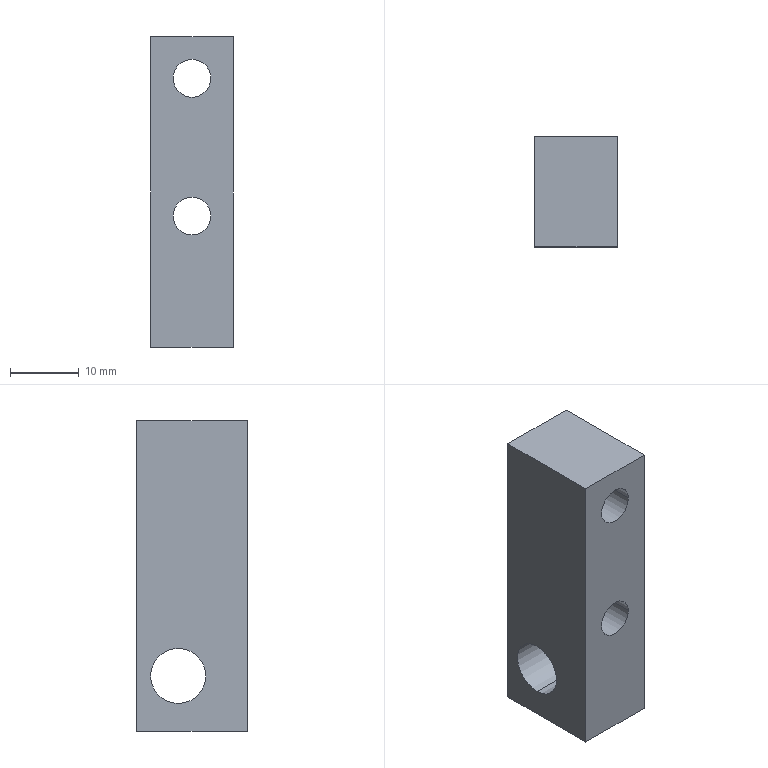Component | SolidWorks | STB-08-008-3 | 1 solid | 12 faces | box 12 x 16 x 45 mm | volume 7277 mm3 | cylinder 6 | plane 6 | commonest cylinder face diameters 5.5 x4 8 x2
build123d program:
from build123d import *

# Parameters (mm, degrees)
SKETCH1_W                  = 45
SKETCH1_H                  = 16
BOSS_EXTRUDE1_DEPTH        = 6
CUT_EXTRUDE1_REACH         = 28.725
SKETCH2_R                  = 4
F_5_5_5_5_DIAMETER_HOLE1_D = 5.5


with BuildPart() as part:
    # Sketch1 → Boss-Extrude1 (new, symmetric)
    with BuildSketch(Plane.XY):
        Rectangle(SKETCH1_W, SKETCH1_H)
    extrude(amount=BOSS_EXTRUDE1_DEPTH, both=True)

    # Sketch2 → Cut-Extrude1 (cut, up to next)
    with BuildSketch(Plane(origin=(0, 0, -6), x_dir=(-1, 0, 0), z_dir=(0, 0, -1)), mode=Mode.PRIVATE) as cut_extrude1_sk1:
        with Locations((14.5, 2)):
            Circle(SKETCH2_R)
    cut_extrude1_tool1 = extrude(cut_extrude1_sk1.sketch, amount=-CUT_EXTRUDE1_REACH, mode=Mode.PRIVATE) & part.part
    add(cut_extrude1_tool1.solids().sort_by_distance((-14.5, 2, -6))[0], mode=Mode.SUBTRACT)

    # 5.5 _5.5_ Diameter Hole1 (through all)
    with Locations(Plane(origin=(0, 8, 0), x_dir=(-1, 0, 0), z_dir=(0, 1, 0))):
        with Locations((-16.5, 0), (3.5, 0)):
            Hole(F_5_5_5_5_DIAMETER_HOLE1_D / 2)


solid = part.part

# Placed as in the assembly
solid = solid.moved(Location((-232.904, 163.999, -4.5), (0, -90, 0)))
STEP:
#1=CARTESIAN_POINT('',(-9.061,6.142,0.4724));
#2=VERTEX_POINT('',#1);
#3=CARTESIAN_POINT('',(-9.278,6.142,0.4724));
#4=VERTEX_POINT('',#3);
#5=CARTESIAN_POINT('',(-9.169,6.142,0.4724));
#6=DIRECTION('',(0.,1.,-0.));
#7=DIRECTION('',(0.,0.,-1.));
#8=AXIS2_PLACEMENT_3D('',#5,#6,#7);
#9=CIRCLE('',#8,0.1083);
#10=EDGE_CURVE('',#2,#4,#9,.T.);
#11=ORIENTED_EDGE('',*,*,#10,.F.);
#12=CARTESIAN_POINT('',(-9.061,6.772,0.4724));
#13=VERTEX_POINT('',#12);
#14=CARTESIAN_POINT('',(-9.061,6.772,0.4724));
#15=DIRECTION('',(0.,1.,0.));
#16=VECTOR('',#15,39.37);
#17=LINE('',#14,#16);
#18=EDGE_CURVE('',#2,#13,#17,.T.);
#19=ORIENTED_EDGE('',*,*,#18,.T.);
#20=CARTESIAN_POINT('',(-9.278,6.772,0.4724));
#21=VERTEX_POINT('',#20);
#22=CARTESIAN_POINT('',(-9.169,6.772,0.4724));
#23=DIRECTION('',(0.,1.,0.));
#24=DIRECTION('',(-1.,0.,-0.));
#25=AXIS2_PLACEMENT_3D('',#22,#23,#24);
#26=CIRCLE('',#25,0.1083);
#27=EDGE_CURVE('',#13,#21,#26,.T.);
#28=ORIENTED_EDGE('',*,*,#27,.T.);
#29=CARTESIAN_POINT('',(-9.278,6.772,0.4724));
#30=DIRECTION('',(0.,1.,0.));
#31=VECTOR('',#30,39.37);
#32=LINE('',#29,#31);
#33=EDGE_CURVE('',#4,#21,#32,.T.);
#34=ORIENTED_EDGE('',*,*,#33,.F.);
#35=EDGE_LOOP('',(#11,#19,#28,#34));
#36=FACE_OUTER_BOUND('',#35,.T.);
#37=CARTESIAN_POINT('',(-9.169,6.772,0.4724));
#38=DIRECTION('',(0.,1.,0.));
#39=DIRECTION('',(-1.,0.,-0.));
#40=AXIS2_PLACEMENT_3D('',#37,#38,#39);
#41=CYLINDRICAL_SURFACE('',#40,0.1083);
#42=ADVANCED_FACE('',(#36),#41,.F.);
#43=CARTESIAN_POINT('',(-9.061,6.142,-0.315));
#44=VERTEX_POINT('',#43);
#45=CARTESIAN_POINT('',(-9.278,6.142,-0.315));
#46=VERTEX_POINT('',#45);
#47=CARTESIAN_POINT('',(-9.169,6.142,-0.315));
#48=DIRECTION('',(0.,1.,-0.));
#49=DIRECTION('',(0.,0.,-1.));
#50=AXIS2_PLACEMENT_3D('',#47,#48,#49);
#51=CIRCLE('',#50,0.1083);
#52=EDGE_CURVE('',#44,#46,#51,.T.);
#53=ORIENTED_EDGE('',*,*,#52,.F.);
#54=CARTESIAN_POINT('',(-9.061,6.772,-0.315));
#55=VERTEX_POINT('',#54);
#56=CARTESIAN_POINT('',(-9.061,6.772,-0.315));
#57=DIRECTION('',(0.,1.,0.));
#58=VECTOR('',#57,39.37);
#59=LINE('',#56,#58);
#60=EDGE_CURVE('',#44,#55,#59,.T.);
#61=ORIENTED_EDGE('',*,*,#60,.T.);
#62=CARTESIAN_POINT('',(-9.278,6.772,-0.315));
#63=VERTEX_POINT('',#62);
#64=CARTESIAN_POINT('',(-9.169,6.772,-0.315));
#65=DIRECTION('',(0.,1.,0.));
#66=DIRECTION('',(-1.,0.,-0.));
#67=AXIS2_PLACEMENT_3D('',#64,#65,#66);
#68=CIRCLE('',#67,0.1083);
#69=EDGE_CURVE('',#55,#63,#68,.T.);
#70=ORIENTED_EDGE('',*,*,#69,.T.);
#71=CARTESIAN_POINT('',(-9.278,6.772,-0.315));
#72=DIRECTION('',(0.,1.,0.));
#73=VECTOR('',#72,39.37);
#74=LINE('',#71,#73);
#75=EDGE_CURVE('',#46,#63,#74,.T.);
#76=ORIENTED_EDGE('',*,*,#75,.F.);
#77=EDGE_LOOP('',(#53,#61,#70,#76));
#78=FACE_OUTER_BOUND('',#77,.T.);
#79=CARTESIAN_POINT('',(-9.169,6.772,-0.315));
#80=DIRECTION('',(0.,1.,0.));
#81=DIRECTION('',(-1.,0.,-0.));
#82=AXIS2_PLACEMENT_3D('',#79,#80,#81);
#83=CYLINDRICAL_SURFACE('',#82,0.1083);
#84=ADVANCED_FACE('',(#78),#83,.F.);
#85=CARTESIAN_POINT('',(-9.406,6.535,-0.5906));
#86=VERTEX_POINT('',#85);
#87=CARTESIAN_POINT('',(-9.406,6.535,-0.9055));
#88=VERTEX_POINT('',#87);
#89=CARTESIAN_POINT('',(-9.406,6.535,-0.748));
#90=DIRECTION('',(1.,0.,0.));
#91=DIRECTION('',(0.,0.,1.));
#92=AXIS2_PLACEMENT_3D('',#89,#90,#91);
#93=CIRCLE('',#92,0.1575);
#94=EDGE_CURVE('',#86,#88,#93,.T.);
#95=ORIENTED_EDGE('',*,*,#94,.F.);
#96=CARTESIAN_POINT('',(-8.933,6.535,-0.5906));
#97=VERTEX_POINT('',#96);
#98=CARTESIAN_POINT('',(-9.406,6.535,-0.5906));
#99=DIRECTION('',(1.,0.,0.));
#100=VECTOR('',#99,39.37);
#101=LINE('',#98,#100);
#102=EDGE_CURVE('',#86,#97,#101,.T.);
#103=ORIENTED_EDGE('',*,*,#102,.T.);
#104=CARTESIAN_POINT('',(-8.933,6.535,-0.9055));
#105=VERTEX_POINT('',#104);
#106=CARTESIAN_POINT('',(-8.933,6.535,-0.748));
#107=DIRECTION('',(1.,0.,0.));
#108=DIRECTION('',(0.,0.,-1.));
#109=AXIS2_PLACEMENT_3D('',#106,#107,#108);
#110=CIRCLE('',#109,0.1575);
#111=EDGE_CURVE('',#97,#105,#110,.T.);
#112=ORIENTED_EDGE('',*,*,#111,.T.);
#113=CARTESIAN_POINT('',(-9.406,6.535,-0.9055));
#114=DIRECTION('',(1.,0.,0.));
#115=VECTOR('',#114,39.37);
#116=LINE('',#113,#115);
#117=EDGE_CURVE('',#88,#105,#116,.T.);
#118=ORIENTED_EDGE('',*,*,#117,.F.);
#119=EDGE_LOOP('',(#95,#103,#112,#118));
#120=FACE_OUTER_BOUND('',#119,.T.);
#121=CARTESIAN_POINT('',(-9.406,6.535,-0.748));
#122=DIRECTION('',(1.,0.,0.));
#123=DIRECTION('',(0.,0.,-1.));
#124=AXIS2_PLACEMENT_3D('',#121,#122,#123);
#125=CYLINDRICAL_SURFACE('',#124,0.1575);
#126=ADVANCED_FACE('',(#120),#125,.F.);
#127=CARTESIAN_POINT('',(-8.933,6.772,-1.063));
#128=VERTEX_POINT('',#127);
#129=CARTESIAN_POINT('',(-8.933,6.142,-1.063));
#130=VERTEX_POINT('',#129);
#131=CARTESIAN_POINT('',(-8.933,6.772,-1.063));
#132=DIRECTION('',(-0.,-1.,-0.));
#133=VECTOR('',#132,39.37);
#134=LINE('',#131,#133);
#135=EDGE_CURVE('',#128,#130,#134,.T.);
#136=ORIENTED_EDGE('',*,*,#135,.T.);
#137=CARTESIAN_POINT('',(-9.406,6.142,-1.063));
#138=VERTEX_POINT('',#137);
#139=CARTESIAN_POINT('',(-9.406,6.142,-1.063));
#140=DIRECTION('',(1.,0.,0.));
#141=VECTOR('',#140,39.37);
#142=LINE('',#139,#141);
#143=EDGE_CURVE('',#138,#130,#142,.T.);
#144=ORIENTED_EDGE('',*,*,#143,.F.);
#145=CARTESIAN_POINT('',(-9.406,6.772,-1.063));
#146=VERTEX_POINT('',#145);
#147=CARTESIAN_POINT('',(-9.406,6.772,-1.063));
#148=DIRECTION('',(-0.,-1.,-0.));
#149=VECTOR('',#148,39.37);
#150=LINE('',#147,#149);
#151=EDGE_CURVE('',#146,#138,#150,.T.);
#152=ORIENTED_EDGE('',*,*,#151,.F.);
#153=CARTESIAN_POINT('',(-9.406,6.772,-1.063));
#154=DIRECTION('',(1.,0.,0.));
#155=VECTOR('',#154,39.37);
#156=LINE('',#153,#155);
#157=EDGE_CURVE('',#146,#128,#156,.T.);
#158=ORIENTED_EDGE('',*,*,#157,.T.);
#159=EDGE_LOOP('',(#136,#144,#152,#158));
#160=FACE_OUTER_BOUND('',#159,.T.);
#161=CARTESIAN_POINT('',(-9.406,6.772,-1.063));
#162=DIRECTION('',(-0.,-0.,1.));
#163=DIRECTION('',(1.,0.,0.));
#164=AXIS2_PLACEMENT_3D('',#161,#162,#163);
#165=PLANE('',#164);
#166=ADVANCED_FACE('',(#160),#165,.F.);
#167=CARTESIAN_POINT('',(-9.169,6.142,0.4724));
#168=DIRECTION('',(0.,1.,-0.));
#169=DIRECTION('',(0.,0.,-1.));
#170=AXIS2_PLACEMENT_3D('',#167,#168,#169);
#171=CIRCLE('',#170,0.1083);
#172=EDGE_CURVE('',#4,#2,#171,.T.);
#173=ORIENTED_EDGE('',*,*,#172,.T.);
#174=ORIENTED_EDGE('',*,*,#10,.T.);
#175=EDGE_LOOP('',(#173,#174));
#176=FACE_BOUND('',#175,.T.);
#177=CARTESIAN_POINT('',(-9.169,6.142,-0.315));
#178=DIRECTION('',(0.,1.,-0.));
#179=DIRECTION('',(0.,0.,-1.));
#180=AXIS2_PLACEMENT_3D('',#177,#178,#179);
#181=CIRCLE('',#180,0.1083);
#182=EDGE_CURVE('',#46,#44,#181,.T.);
#183=ORIENTED_EDGE('',*,*,#182,.T.);
#184=ORIENTED_EDGE('',*,*,#52,.T.);
#185=EDGE_LOOP('',(#183,#184));
#186=FACE_BOUND('',#185,.T.);
#187=CARTESIAN_POINT('',(-8.933,6.142,0.7087));
#188=VERTEX_POINT('',#187);
#189=CARTESIAN_POINT('',(-8.933,6.142,-1.063));
#190=DIRECTION('',(-0.,-0.,1.));
#191=VECTOR('',#190,39.37);
#192=LINE('',#189,#191);
#193=EDGE_CURVE('',#130,#188,#192,.T.);
#194=ORIENTED_EDGE('',*,*,#193,.T.);
#195=CARTESIAN_POINT('',(-9.406,6.142,0.7087));
#196=VERTEX_POINT('',#195);
#197=CARTESIAN_POINT('',(-9.406,6.142,0.7087));
#198=DIRECTION('',(1.,0.,0.));
#199=VECTOR('',#198,39.37);
#200=LINE('',#197,#199);
#201=EDGE_CURVE('',#196,#188,#200,.T.);
#202=ORIENTED_EDGE('',*,*,#201,.F.);
#203=CARTESIAN_POINT('',(-9.406,6.142,-1.063));
#204=DIRECTION('',(-0.,-0.,1.));
#205=VECTOR('',#204,39.37);
#206=LINE('',#203,#205);
#207=EDGE_CURVE('',#138,#196,#206,.T.);
#208=ORIENTED_EDGE('',*,*,#207,.F.);
#209=ORIENTED_EDGE('',*,*,#143,.T.);
#210=EDGE_LOOP('',(#194,#202,#208,#209));
#211=FACE_OUTER_BOUND('',#210,.T.);
#212=CARTESIAN_POINT('',(-9.406,6.142,-1.063));
#213=DIRECTION('',(0.,1.,0.));
#214=DIRECTION('',(0.,0.,-1.));
#215=AXIS2_PLACEMENT_3D('',#212,#213,#214);
#216=PLANE('',#215);
#217=ADVANCED_FACE('',(#176,#186,#211),#216,.F.);
#218=CARTESIAN_POINT('',(-8.933,6.772,0.7087));
#219=VERTEX_POINT('',#218);
#220=CARTESIAN_POINT('',(-8.933,6.772,0.7087));
#221=DIRECTION('',(0.,1.,0.));
#222=VECTOR('',#221,39.37);
#223=LINE('',#220,#222);
#224=EDGE_CURVE('',#188,#219,#223,.T.);
#225=ORIENTED_EDGE('',*,*,#224,.T.);
#226=CARTESIAN_POINT('',(-9.406,6.772,0.7087));
#227=VERTEX_POINT('',#226);
#228=CARTESIAN_POINT('',(-9.406,6.772,0.7087));
#229=DIRECTION('',(1.,0.,0.));
#230=VECTOR('',#229,39.37);
#231=LINE('',#228,#230);
#232=EDGE_CURVE('',#227,#219,#231,.T.);
#233=ORIENTED_EDGE('',*,*,#232,.F.);
#234=CARTESIAN_POINT('',(-9.406,6.772,0.7087));
#235=DIRECTION('',(0.,1.,0.));
#236=VECTOR('',#235,39.37);
#237=LINE('',#234,#236);
#238=EDGE_CURVE('',#196,#227,#237,.T.);
#239=ORIENTED_EDGE('',*,*,#238,.F.);
#240=ORIENTED_EDGE('',*,*,#201,.T.);
#241=EDGE_LOOP('',(#225,#233,#239,#240));
#242=FACE_OUTER_BOUND('',#241,.T.);
#243=CARTESIAN_POINT('',(-9.406,6.772,0.7087));
#244=DIRECTION('',(0.,0.,-1.));
#245=DIRECTION('',(-1.,-0.,-0.));
#246=AXIS2_PLACEMENT_3D('',#243,#244,#245);
#247=PLANE('',#246);
#248=ADVANCED_FACE('',(#242),#247,.F.);
#249=CARTESIAN_POINT('',(-9.169,6.772,0.4724));
#250=DIRECTION('',(0.,1.,0.));
#251=DIRECTION('',(-1.,0.,-0.));
#252=AXIS2_PLACEMENT_3D('',#249,#250,#251);
#253=CIRCLE('',#252,0.1083);
#254=EDGE_CURVE('',#21,#13,#253,.T.);
#255=ORIENTED_EDGE('',*,*,#254,.F.);
#256=ORIENTED_EDGE('',*,*,#27,.F.);
#257=EDGE_LOOP('',(#255,#256));
#258=FACE_BOUND('',#257,.T.);
#259=CARTESIAN_POINT('',(-9.169,6.772,-0.315));
#260=DIRECTION('',(0.,1.,0.));
#261=DIRECTION('',(-1.,0.,-0.));
#262=AXIS2_PLACEMENT_3D('',#259,#260,#261);
#263=CIRCLE('',#262,0.1083);
#264=EDGE_CURVE('',#63,#55,#263,.T.);
#265=ORIENTED_EDGE('',*,*,#264,.F.);
#266=ORIENTED_EDGE('',*,*,#69,.F.);
#267=EDGE_LOOP('',(#265,#266));
#268=FACE_BOUND('',#267,.T.);
#269=CARTESIAN_POINT('',(-8.933,6.772,-1.063));
#270=DIRECTION('',(0.,0.,-1.));
#271=VECTOR('',#270,39.37);
#272=LINE('',#269,#271);
#273=EDGE_CURVE('',#219,#128,#272,.T.);
#274=ORIENTED_EDGE('',*,*,#273,.T.);
#275=ORIENTED_EDGE('',*,*,#157,.F.);
#276=CARTESIAN_POINT('',(-9.406,6.772,-1.063));
#277=DIRECTION('',(0.,0.,-1.));
#278=VECTOR('',#277,39.37);
#279=LINE('',#276,#278);
#280=EDGE_CURVE('',#227,#146,#279,.T.);
#281=ORIENTED_EDGE('',*,*,#280,.F.);
#282=ORIENTED_EDGE('',*,*,#232,.T.);
#283=EDGE_LOOP('',(#274,#275,#281,#282));
#284=FACE_OUTER_BOUND('',#283,.T.);
#285=CARTESIAN_POINT('',(-9.406,6.772,-1.063));
#286=DIRECTION('',(0.,-1.,-0.));
#287=DIRECTION('',(1.,0.,0.));
#288=AXIS2_PLACEMENT_3D('',#285,#286,#287);
#289=PLANE('',#288);
#290=ADVANCED_FACE('',(#258,#268,#284),#289,.F.);
#291=CARTESIAN_POINT('',(-9.406,6.535,-0.748));
#292=DIRECTION('',(1.,0.,0.));
#293=DIRECTION('',(0.,0.,1.));
#294=AXIS2_PLACEMENT_3D('',#291,#292,#293);
#295=CIRCLE('',#294,0.1575);
#296=EDGE_CURVE('',#88,#86,#295,.T.);
#297=ORIENTED_EDGE('',*,*,#296,.T.);
#298=ORIENTED_EDGE('',*,*,#94,.T.);
#299=EDGE_LOOP('',(#297,#298));
#300=FACE_BOUND('',#299,.T.);
#301=ORIENTED_EDGE('',*,*,#151,.T.);
#302=ORIENTED_EDGE('',*,*,#207,.T.);
#303=ORIENTED_EDGE('',*,*,#238,.T.);
#304=ORIENTED_EDGE('',*,*,#280,.T.);
#305=EDGE_LOOP('',(#301,#302,#303,#304));
#306=FACE_OUTER_BOUND('',#305,.T.);
#307=CARTESIAN_POINT('',(-9.406,6.142,-1.063));
#308=DIRECTION('',(-1.,-0.,-0.));
#309=DIRECTION('',(-0.,-0.,1.));
#310=AXIS2_PLACEMENT_3D('',#307,#308,#309);
#311=PLANE('',#310);
#312=ADVANCED_FACE('',(#300,#306),#311,.T.);
#313=CARTESIAN_POINT('',(-8.933,6.535,-0.748));
#314=DIRECTION('',(1.,0.,0.));
#315=DIRECTION('',(0.,0.,-1.));
#316=AXIS2_PLACEMENT_3D('',#313,#314,#315);
#317=CIRCLE('',#316,0.1575);
#318=EDGE_CURVE('',#105,#97,#317,.T.);
#319=ORIENTED_EDGE('',*,*,#318,.F.);
#320=ORIENTED_EDGE('',*,*,#111,.F.);
#321=EDGE_LOOP('',(#319,#320));
#322=FACE_BOUND('',#321,.T.);
#323=ORIENTED_EDGE('',*,*,#135,.F.);
#324=ORIENTED_EDGE('',*,*,#273,.F.);
#325=ORIENTED_EDGE('',*,*,#224,.F.);
#326=ORIENTED_EDGE('',*,*,#193,.F.);
#327=EDGE_LOOP('',(#323,#324,#325,#326));
#328=FACE_OUTER_BOUND('',#327,.T.);
#329=CARTESIAN_POINT('',(-8.933,6.142,-1.063));
#330=DIRECTION('',(-1.,-0.,-0.));
#331=DIRECTION('',(-0.,-0.,1.));
#332=AXIS2_PLACEMENT_3D('',#329,#330,#331);
#333=PLANE('',#332);
#334=ADVANCED_FACE('',(#322,#328),#333,.F.);
#335=ORIENTED_EDGE('',*,*,#102,.F.);
#336=ORIENTED_EDGE('',*,*,#296,.F.);
#337=ORIENTED_EDGE('',*,*,#117,.T.);
#338=ORIENTED_EDGE('',*,*,#318,.T.);
#339=EDGE_LOOP('',(#335,#336,#337,#338));
#340=FACE_OUTER_BOUND('',#339,.T.);
#341=CARTESIAN_POINT('',(-9.406,6.535,-0.748));
#342=DIRECTION('',(1.,0.,0.));
#343=DIRECTION('',(0.,0.,-1.));
#344=AXIS2_PLACEMENT_3D('',#341,#342,#343);
#345=CYLINDRICAL_SURFACE('',#344,0.1575);
#346=ADVANCED_FACE('',(#340),#345,.F.);
#347=ORIENTED_EDGE('',*,*,#60,.F.);
#348=ORIENTED_EDGE('',*,*,#182,.F.);
#349=ORIENTED_EDGE('',*,*,#75,.T.);
#350=ORIENTED_EDGE('',*,*,#264,.T.);
#351=EDGE_LOOP('',(#347,#348,#349,#350));
#352=FACE_OUTER_BOUND('',#351,.T.);
#353=CARTESIAN_POINT('',(-9.169,6.772,-0.315));
#354=DIRECTION('',(0.,1.,0.));
#355=DIRECTION('',(-1.,0.,-0.));
#356=AXIS2_PLACEMENT_3D('',#353,#354,#355);
#357=CYLINDRICAL_SURFACE('',#356,0.1083);
#358=ADVANCED_FACE('',(#352),#357,.F.);
#359=ORIENTED_EDGE('',*,*,#18,.F.);
#360=ORIENTED_EDGE('',*,*,#172,.F.);
#361=ORIENTED_EDGE('',*,*,#33,.T.);
#362=ORIENTED_EDGE('',*,*,#254,.T.);
#363=EDGE_LOOP('',(#359,#360,#361,#362));
#364=FACE_OUTER_BOUND('',#363,.T.);
#365=CARTESIAN_POINT('',(-9.169,6.772,0.4724));
#366=DIRECTION('',(0.,1.,0.));
#367=DIRECTION('',(-1.,0.,-0.));
#368=AXIS2_PLACEMENT_3D('',#365,#366,#367);
#369=CYLINDRICAL_SURFACE('',#368,0.1083);
#370=ADVANCED_FACE('',(#364),#369,.F.);
#371=CLOSED_SHELL('',(#42,#84,#126,#166,#217,#248,#290,#312,#334,#346,#358,#370));
#372=MANIFOLD_SOLID_BREP('',#371);
#373=CARTESIAN_POINT('',(0.,0.,0.));
#374=DIRECTION('',(0.,0.,1.));
#375=DIRECTION('',(1.,0.,0.));
#376=AXIS2_PLACEMENT_3D('',#373,#374,#375);
#377=(LENGTH_UNIT()NAMED_UNIT(*)SI_UNIT($,.METRE.));
#378=LENGTH_MEASURE_WITH_UNIT(LENGTH_MEASURE(0.0254),#377);
#379=DIMENSIONAL_EXPONENTS(1.,0.,0.,0.,0.,0.,0.);
#380=(CONVERSION_BASED_UNIT('',#378)LENGTH_UNIT()NAMED_UNIT(#379));
#381=UNCERTAINTY_MEASURE_WITH_UNIT(LENGTH_MEASURE(0.00001),#380,'','');
#382=(NAMED_UNIT(*)PLANE_ANGLE_UNIT()SI_UNIT($,.RADIAN.));
#383=(NAMED_UNIT(*)SI_UNIT($,.STERADIAN.)SOLID_ANGLE_UNIT());
#384=(GEOMETRIC_REPRESENTATION_CONTEXT(3)GLOBAL_UNCERTAINTY_ASSIGNED_CONTEXT((#381))GLOBAL_UNIT_ASSIGNED_CONTEXT((#380,#382,#383))REPRESENTATION_CONTEXT('',''));
#385=ADVANCED_BREP_SHAPE_REPRESENTATION('',(#372,#376),#384);
#386=COLOUR_RGB('',0.7922,0.8196,0.9333);
#387=FILL_AREA_STYLE_COLOUR('',#386);
#388=FILL_AREA_STYLE('',(#387));
#389=SURFACE_STYLE_FILL_AREA(#388);
#390=SURFACE_SIDE_STYLE('',(#389));
#391=SURFACE_STYLE_USAGE(.BOTH.,#390);
#392=PRESENTATION_STYLE_ASSIGNMENT((#391));
#393=STYLED_ITEM('',(#392),#372);
#394=(LENGTH_UNIT()NAMED_UNIT(*)SI_UNIT($,.METRE.));
#395=LENGTH_MEASURE_WITH_UNIT(LENGTH_MEASURE(0.0254),#394);
#396=DIMENSIONAL_EXPONENTS(1.,0.,0.,0.,0.,0.,0.);
#397=(CONVERSION_BASED_UNIT('',#395)LENGTH_UNIT()NAMED_UNIT(#396));
#398=UNCERTAINTY_MEASURE_WITH_UNIT(LENGTH_MEASURE(0.00001),#397,'','');
#399=(NAMED_UNIT(*)PLANE_ANGLE_UNIT()SI_UNIT($,.RADIAN.));
#400=(NAMED_UNIT(*)SI_UNIT($,.STERADIAN.)SOLID_ANGLE_UNIT());
#401=(GEOMETRIC_REPRESENTATION_CONTEXT(3)GLOBAL_UNCERTAINTY_ASSIGNED_CONTEXT((#398))GLOBAL_UNIT_ASSIGNED_CONTEXT((#397,#399,#400))REPRESENTATION_CONTEXT('',''));
#402=MECHANICAL_DESIGN_GEOMETRIC_PRESENTATION_REPRESENTATION('',(#393),#401);
#403=PRESENTATION_LAYER_ASSIGNMENT('','',(#393));